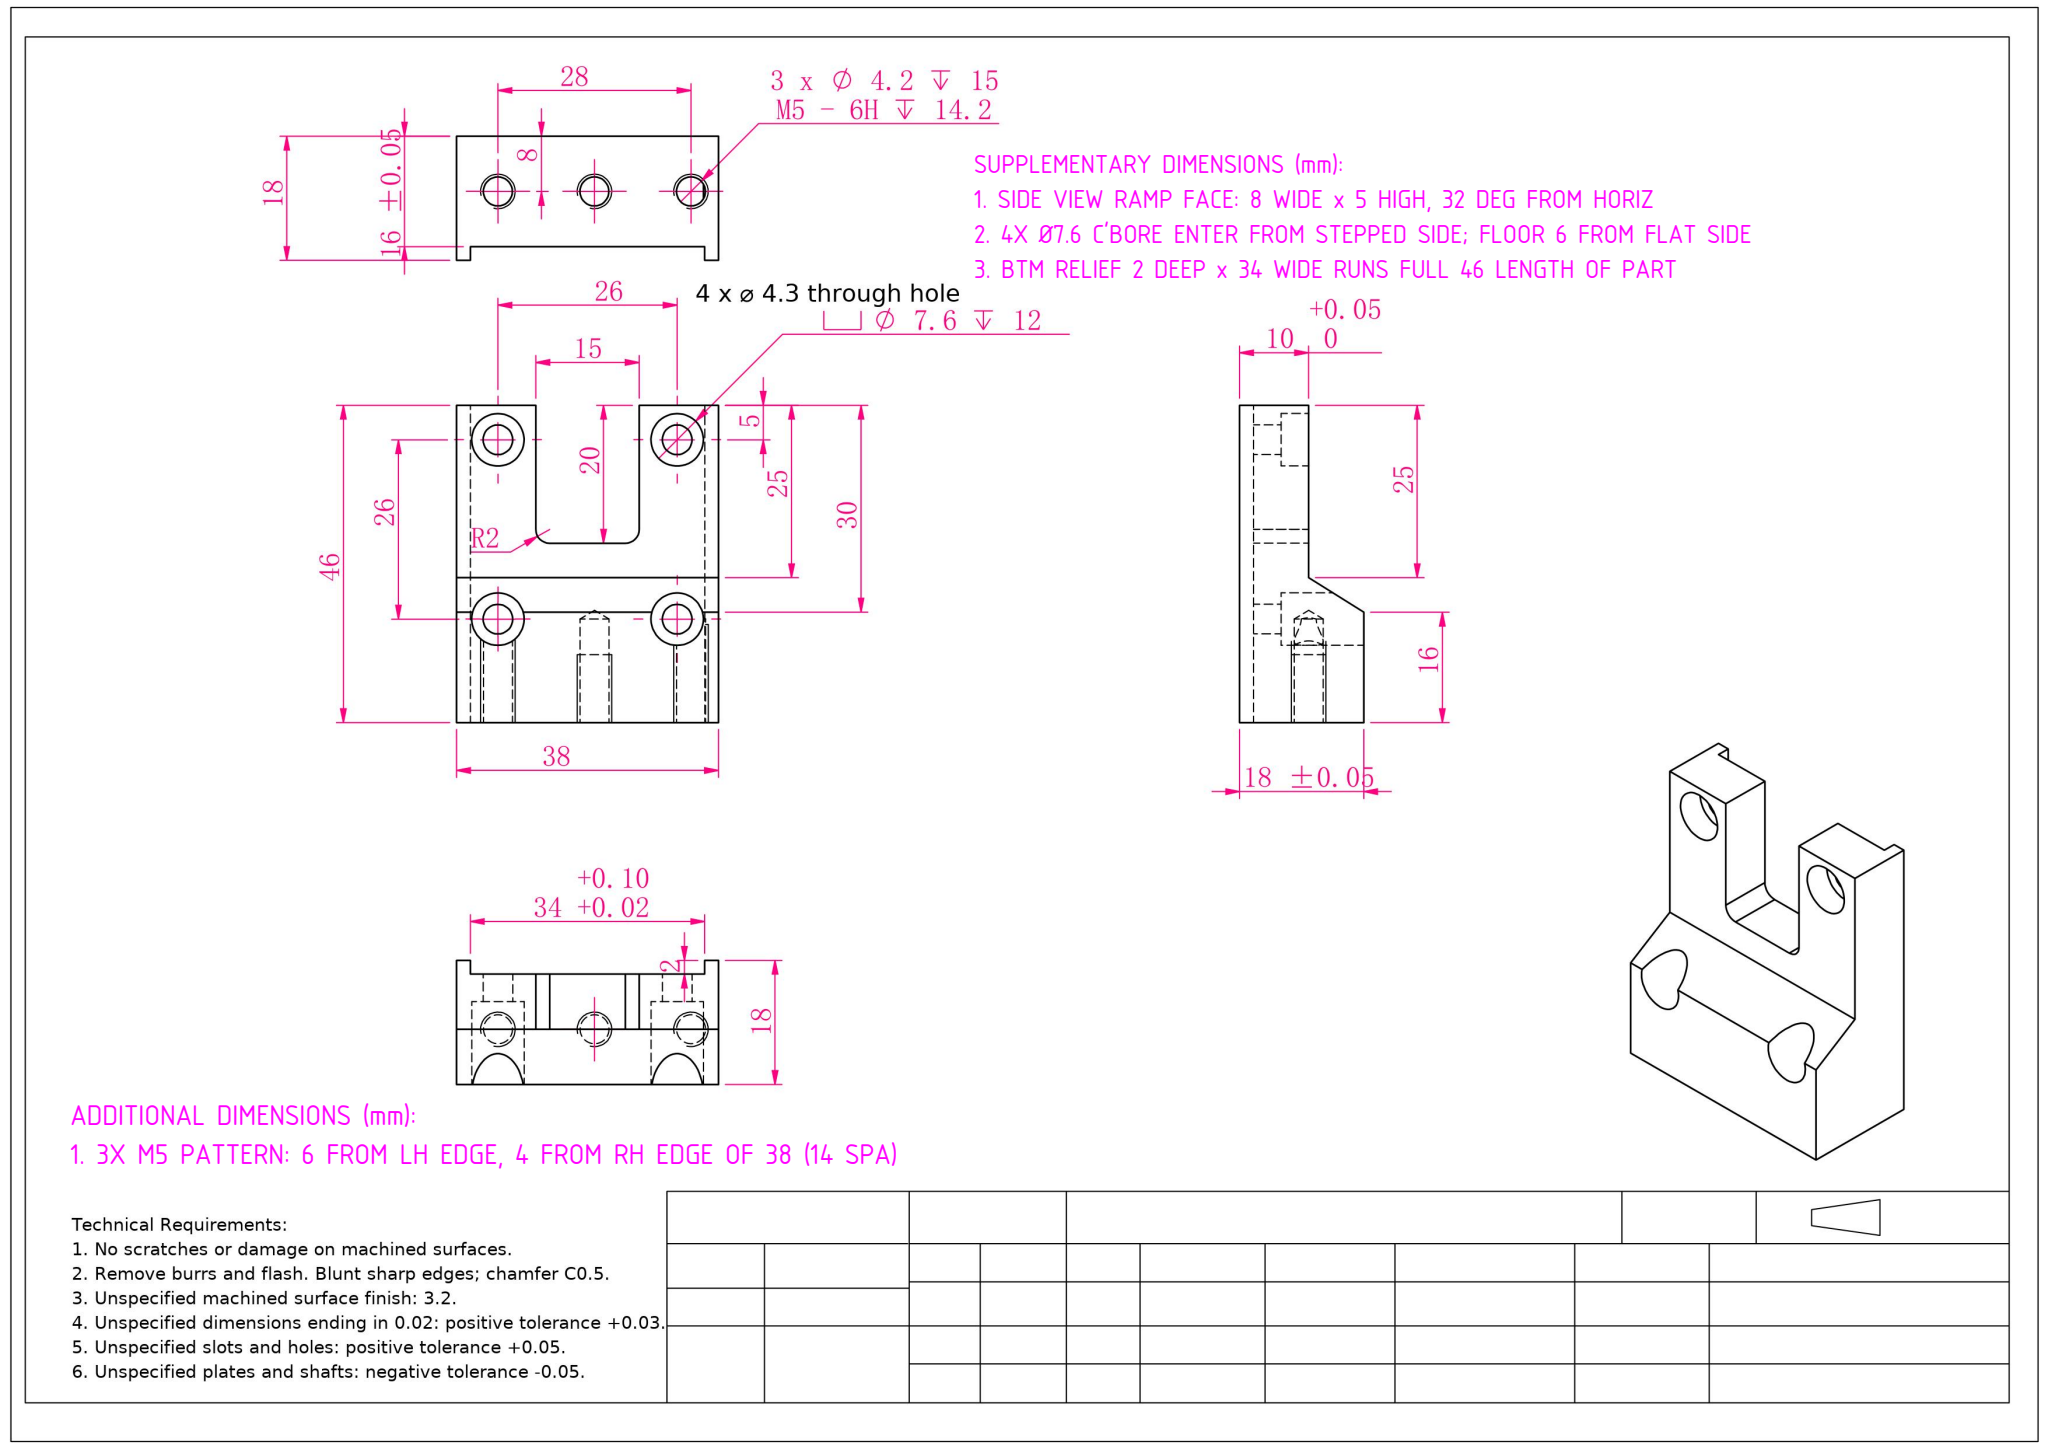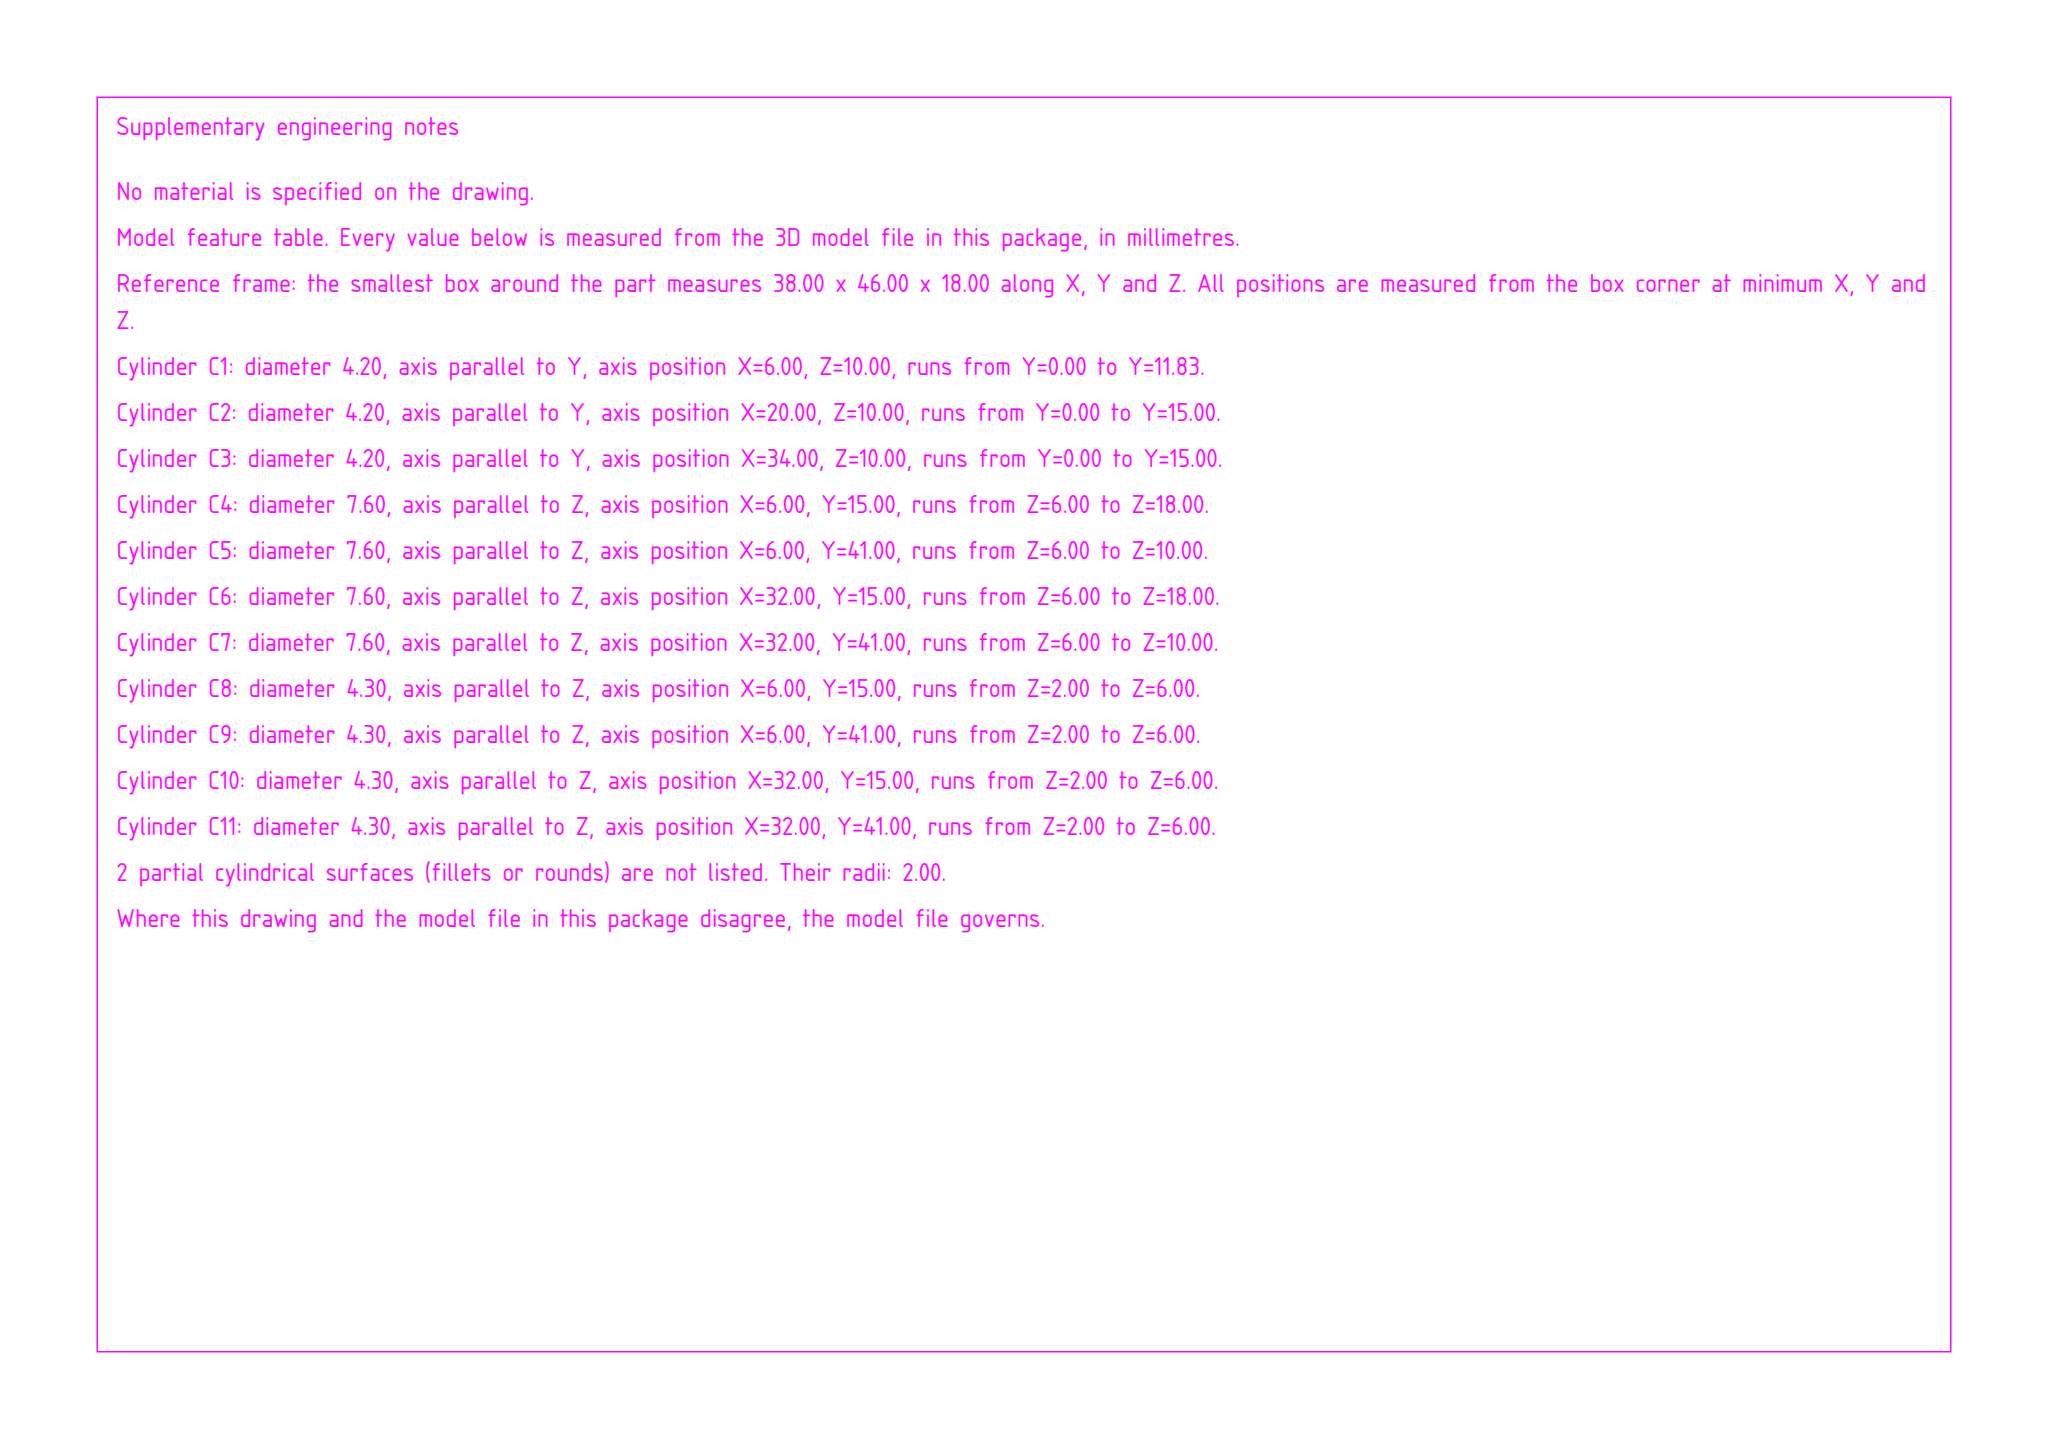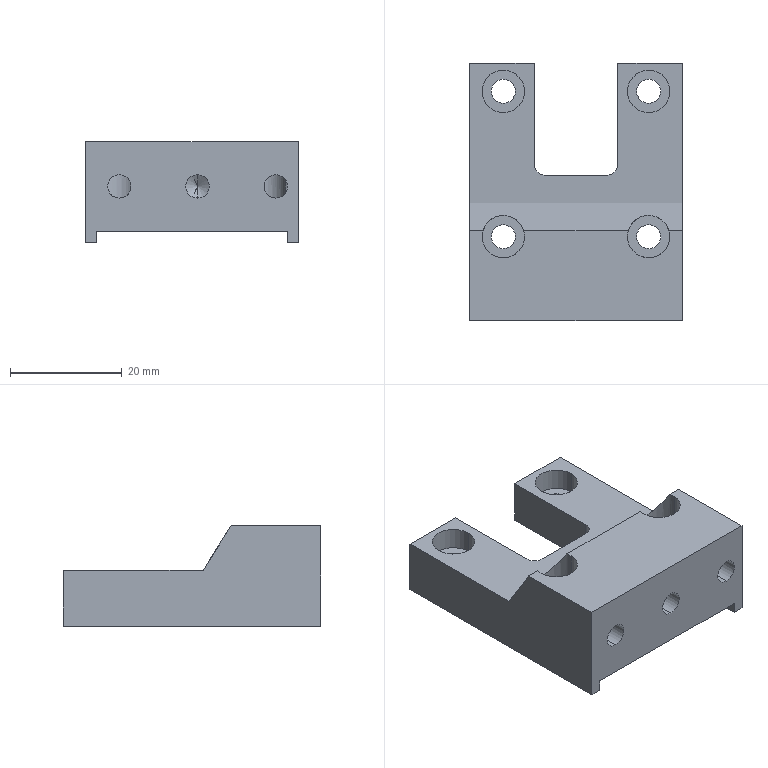Part | SolidWorks | mm | 1 solid | 47 faces | box 38 x 46 x 18 mm | volume 15424 mm3 | cylinder 24 | plane 20 | cone 3 | commonest cylinder face diameters 7.6 x8 4.3 x8 4.2 x6 4 x2
build123d program:
from build123d import *

# Parameters (mm, degrees)
SKETCH1_W                                       = 38
SKETCH1_H                                       = 46
EXTRUDE1_DEPTH                                  = 18
SKETCH2_W                                       = 34
SKETCH2_H                                       = 46
EXTRUDE2_DEPTH                                  = 2
M4_HEX_SOCKET_HEAD_CAP_SCREW_CBORE1_D           = 4.3
M4_HEX_SOCKET_HEAD_CAP_SCREW_CBORE1_CBORE_D     = 7.6
M4_HEX_SOCKET_HEAD_CAP_SCREW_CBORE1_CBORE_DEPTH = 12
M5_TAPPED_HOLE1_D                               = 4.2
M5_TAPPED_HOLE1_DEPTH                           = 15
M5_TAPPED_HOLE1_TIP                             = 1.262
SKETCH9_W                                       = 15
SKETCH9_H                                       = 20
CUT_EXTRUDE2_DEPTH                              = 63.322
FILLET1_R                                       = 2
CUT_EXTRUDE3_DEPTH                              = 63.322


with BuildPart() as part:
    # Sketch1 → Extrude1 (new body)
    with BuildSketch(Plane.XY):
        with Locations((19, 23)):
            Rectangle(SKETCH1_W, SKETCH1_H)
    extrude(amount=EXTRUDE1_DEPTH)

    # Sketch2 → Extrude2 (cut)
    with BuildSketch(Plane(origin=(0, 0, 0), x_dir=(-1, 0, 0), z_dir=(0, 0, -1))):
        with Locations((-19, 23)):
            Rectangle(SKETCH2_W, SKETCH2_H)
    extrude(amount=-EXTRUDE2_DEPTH, mode=Mode.SUBTRACT)

    # M4 Hex Socket Head Cap Screw CBORE1 (through all)
    with Locations(Plane.XY.offset(18)):
        with Locations((6, 15), (6, 41), (32, 41), (32, 15)):
            CounterBoreHole(M4_HEX_SOCKET_HEAD_CAP_SCREW_CBORE1_D / 2, M4_HEX_SOCKET_HEAD_CAP_SCREW_CBORE1_CBORE_D / 2, M4_HEX_SOCKET_HEAD_CAP_SCREW_CBORE1_CBORE_DEPTH)

    # M5 Tapped Hole1
    with Locations(Plane.XZ):
        with Locations((34, 10), (6, 10), (20, 10)):
            Hole(M5_TAPPED_HOLE1_D / 2, depth=M5_TAPPED_HOLE1_DEPTH)
            with Locations((0, 0, -(M5_TAPPED_HOLE1_DEPTH + M5_TAPPED_HOLE1_TIP / 2))):  # 118° drill point
                Cone(0, M5_TAPPED_HOLE1_D / 2, M5_TAPPED_HOLE1_TIP, mode=Mode.SUBTRACT)

    # Sketch9 → Cut-Extrude2 (cut, through all)
    with BuildSketch(Plane.XY.offset(18)):
        with Locations((19, 36)):
            Rectangle(SKETCH9_W, SKETCH9_H)
    extrude(amount=-CUT_EXTRUDE2_DEPTH, mode=Mode.SUBTRACT)

    # Fillet1
    fillet1_edges = [part.edges().sort_by_distance(p)[0] for p in [
        (11.5, 26, 10),
        (26.5, 26, 10),
    ]]
    fillet(fillet1_edges, radius=FILLET1_R)

    # Sketch10 → Cut-Extrude3 (cut, through all)
    with BuildSketch(Plane(origin=(38, 0, 0), x_dir=(0, 0, -1), z_dir=(1, 0, 0))):
        Polygon((-10, 46), (-10, 21), (-18, 16), (-18, 46), align=None)
    extrude(amount=-CUT_EXTRUDE3_DEPTH, mode=Mode.SUBTRACT)


solid = part.part